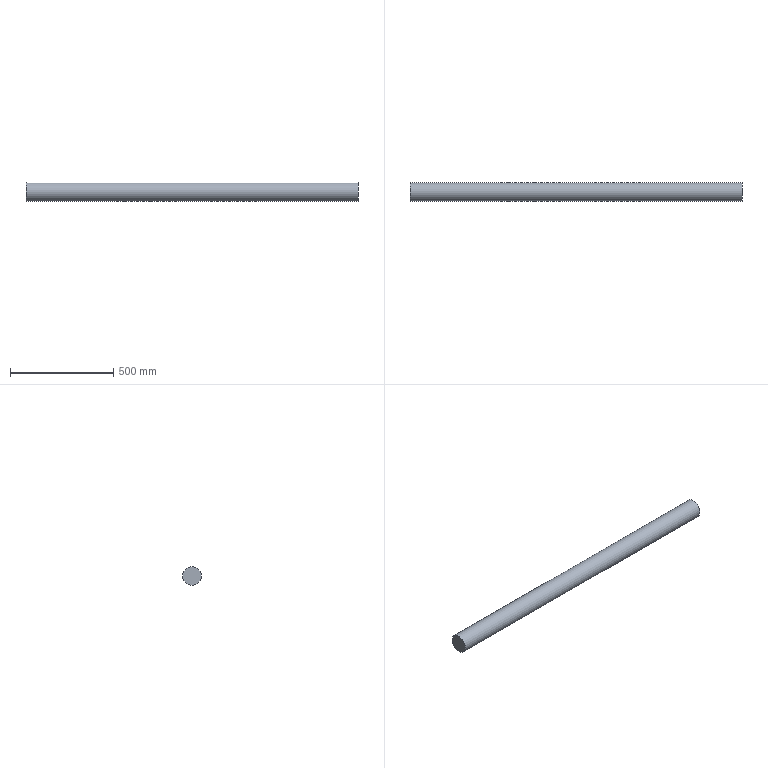Component | NX | SIM15_C_SPINDELANSCHLAG_116 | 1 solid | 3 faces | volume 10210569 mm3 | plane 2 | cylinder 1 | commonest cylinder face diameters 90 x1